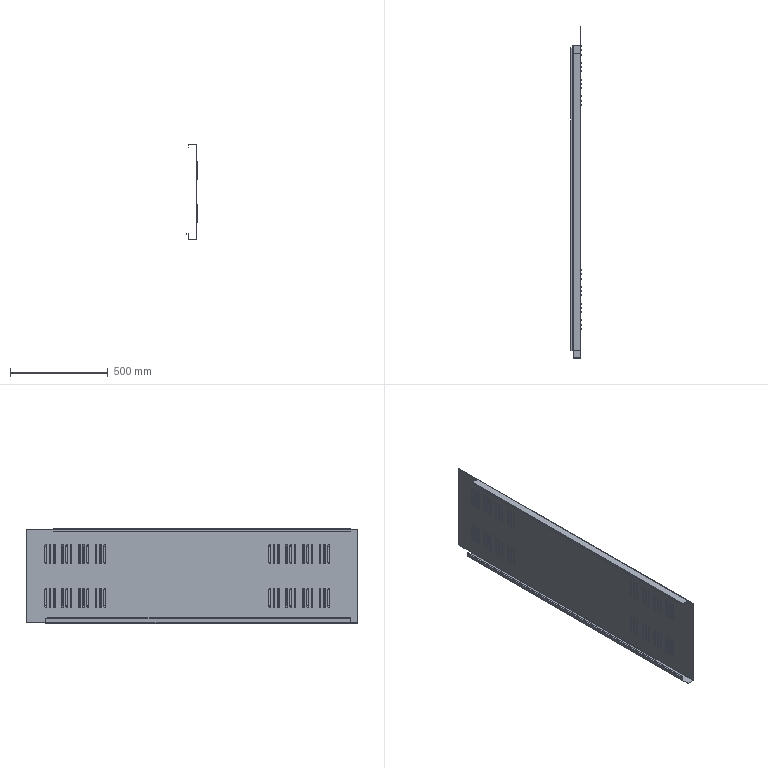Component | SolidWorks | AirFurnaceElectricalCabinet-RightSidePlate-1 | 1 solid | 725 faces | volume 1224972 mm3 | cylinder 202 | torus 192 | sphere 192 | plane 139 | commonest cylinder face diameters 10 x96 7.6 x48 12.4 x48 1.5 x5 3.9 x5